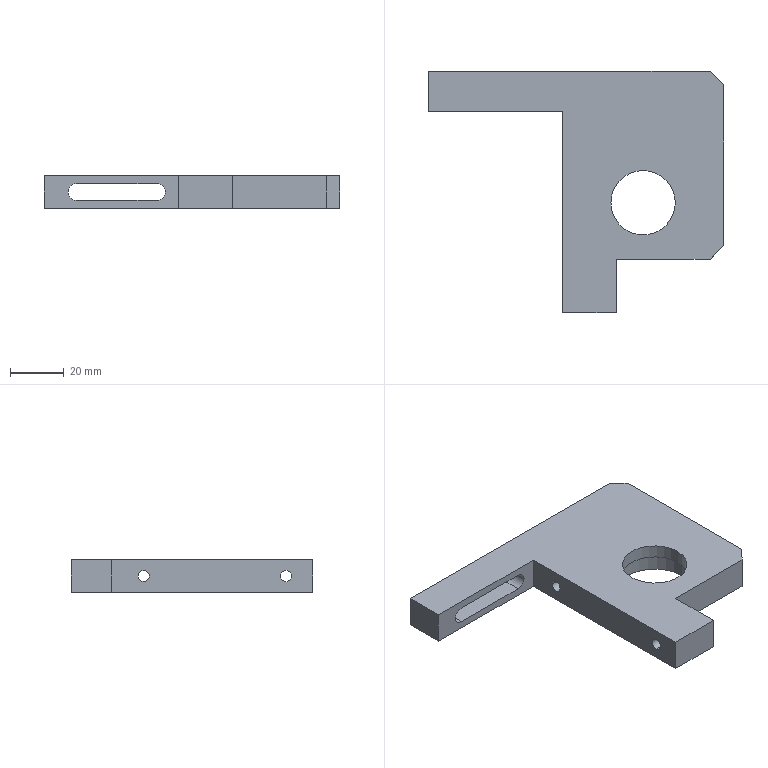Component | SolidWorks | LD101-02--Q1025-Q1-2-1 | 1 solid | 29 faces | box 110 x 90 x 12 mm | volume 50389 mm3 | plane 16 | cylinder 13 | commonest cylinder face diameters 4.2 x4 6.2 x3 10 x2 24 x2 28 x2 | material 45
build123d program:
from build123d import *

# Parameters (mm, degrees)
SKETCH1_W           = 110
SKETCH1_H           = 90
BOSS_EXTRUDE1_DEPTH = 6
SKETCH2_W           = 50
SKETCH2_H           = 75
CUT_EXTRUDE1_DEPTH  = 107.156
SKETCH3_R           = 14
CUT_EXTRUDE2_DEPTH  = 7
SKETCH4_R           = 12
CUT_EXTRUDE3_DEPTH  = 106.707
CUT_EXTRUDE4_DEPTH  = 94.199
SKETCH6_W           = 40
SKETCH6_H           = 20
CUT_EXTRUDE5_DEPTH  = 107.156
M5_TAPPED_HOLE1_D   = 4.2
CHAMFER1_SIZE       = 5
SKETCH9_R           = 5
CUT_EXTRUDE6_DEPTH  = 40
M5_TAPPED_HOLE2_D   = 4.2


with BuildPart() as part:
    # Sketch1 → Boss-Extrude1 (new, symmetric)
    with BuildSketch(Plane(origin=(0, 0, 0), x_dir=(0, 0, -1), z_dir=(1, 0, 0))):
        with Locations((0, 45)):
            Rectangle(SKETCH1_W, SKETCH1_H)
    extrude(amount=BOSS_EXTRUDE1_DEPTH, both=True)

    # Sketch2 → Cut-Extrude1 (cut, through all)
    with BuildSketch(Plane(origin=(6, 0, 0), x_dir=(0, 0, -1), z_dir=(1, 0, 0))):
        with Locations((30, 52.5)):
            Rectangle(SKETCH2_W, SKETCH2_H)
    extrude(amount=-CUT_EXTRUDE1_DEPTH, mode=Mode.SUBTRACT)

    # Sketch3 → Cut-Extrude2 (cut)
    with BuildSketch(Plane.ZY.offset(6)):
        with Locations((25, 49)):
            Circle(SKETCH3_R)
    extrude(amount=-CUT_EXTRUDE2_DEPTH, mode=Mode.SUBTRACT)

    # Sketch4 → Cut-Extrude3 (cut, through all)
    with BuildSketch(Plane.ZY.offset(-1)):
        with Locations((25, 49)):
            Circle(SKETCH4_R)
    extrude(amount=-CUT_EXTRUDE3_DEPTH, mode=Mode.SUBTRACT)

    # Sketch5 → Cut-Extrude4 (cut, through all)
    with BuildSketch(Plane(origin=(0, 15, 0), x_dir=(1, 0, 0), z_dir=(0, 1, 0))):
        with BuildLine():
            Line((3.1, 43), (3.1, 13))
            ThreePointArc((3.1, 13), (0, 9.9), (-3.1, 13))
            Line((-3.1, 13), (-3.1, 43))
            ThreePointArc((-3.1, 43), (0, 46.1), (3.1, 43))
        make_face()
    extrude(amount=-CUT_EXTRUDE4_DEPTH, mode=Mode.SUBTRACT)

    # Sketch6 → Cut-Extrude5 (cut, through all)
    with BuildSketch(Plane.ZY.offset(6)):
        with Locations((35, 80)):
            Rectangle(SKETCH6_W, SKETCH6_H)
    extrude(amount=-CUT_EXTRUDE5_DEPTH, mode=Mode.SUBTRACT)

    # M5 Tapped Hole1 (through all)
    with Locations(Plane(origin=(0, 0, 15), x_dir=(-1, 0, 0), z_dir=(0, 0, 1))):
        with Locations((0, -80)):
            Hole(M5_TAPPED_HOLE1_D / 2)

    # Chamfer1
    chamfer1_edges = [part.edges().sort_by_distance(p)[0] for p in [
        (0, 70, 55),
        (0, 0, 55),
    ]]
    chamfer(chamfer1_edges, length=CHAMFER1_SIZE)

    # Sketch9 → Cut-Extrude6 (cut)
    with BuildSketch(Plane.XY.offset(55)):
        with Locations((0, 27)):
            Circle(SKETCH9_R)
    extrude(amount=-CUT_EXTRUDE6_DEPTH, mode=Mode.SUBTRACT)

    # M5 Tapped Hole2 (through all)
    with Locations(Plane(origin=(0, 0, -5), x_dir=(-1, 0, 0), z_dir=(0, 0, -1))):
        with Locations((0, 27)):
            Hole(M5_TAPPED_HOLE2_D / 2)


solid = part.part

# Placed as in the assembly
solid = solid.moved(Location((346.71, -132.897, 287.257), (180, 90, 0)))
STEP:
#1=COLOUR_RGB('',0.7922,0.8196,0.9333);
#2=FILL_AREA_STYLE_COLOUR('',#1);
#3=FILL_AREA_STYLE('',(#2));
#4=SURFACE_STYLE_FILL_AREA(#3);
#5=SURFACE_SIDE_STYLE('',(#4));
#6=SURFACE_STYLE_USAGE(.BOTH.,#5);
#7=PRESENTATION_STYLE_ASSIGNMENT((#6));
#8=CARTESIAN_POINT('',(14.241,-6.378,11.309));
#9=VERTEX_POINT('',#8);
#10=CARTESIAN_POINT('',(14.241,-6.212,11.309));
#11=VERTEX_POINT('',#10);
#12=CARTESIAN_POINT('',(14.241,-6.295,11.309));
#13=DIRECTION('',(1.,0.,-0.));
#14=DIRECTION('',(0.,1.,0.));
#15=AXIS2_PLACEMENT_3D('',#12,#13,#14);
#16=CIRCLE('',#15,0.08268);
#17=EDGE_CURVE('',#9,#11,#16,.T.);
#18=ORIENTED_EDGE('',*,*,#17,.T.);
#19=CARTESIAN_POINT('',(13.453,-6.212,11.309));
#20=VERTEX_POINT('',#19);
#21=CARTESIAN_POINT('',(13.453,-6.212,11.309));
#22=DIRECTION('',(-1.,-0.,0.));
#23=VECTOR('',#22,39.37);
#24=LINE('',#21,#23);
#25=EDGE_CURVE('',#11,#20,#24,.T.);
#26=ORIENTED_EDGE('',*,*,#25,.T.);
#27=CARTESIAN_POINT('',(13.453,-6.378,11.309));
#28=VERTEX_POINT('',#27);
#29=CARTESIAN_POINT('',(13.453,-6.295,11.309));
#30=DIRECTION('',(-1.,-0.,0.));
#31=DIRECTION('',(0.,-1.,0.));
#32=AXIS2_PLACEMENT_3D('',#29,#30,#31);
#33=CIRCLE('',#32,0.08268);
#34=EDGE_CURVE('',#20,#28,#33,.T.);
#35=ORIENTED_EDGE('',*,*,#34,.T.);
#36=CARTESIAN_POINT('',(13.453,-6.378,11.309));
#37=DIRECTION('',(-1.,-0.,0.));
#38=VECTOR('',#37,39.37);
#39=LINE('',#36,#38);
#40=EDGE_CURVE('',#9,#28,#39,.T.);
#41=ORIENTED_EDGE('',*,*,#40,.F.);
#42=EDGE_LOOP('',(#18,#26,#35,#41));
#43=FACE_OUTER_BOUND('',#42,.T.);
#44=CARTESIAN_POINT('',(13.453,-6.295,11.309));
#45=DIRECTION('',(-1.,-0.,0.));
#46=DIRECTION('',(0.,-1.,0.));
#47=AXIS2_PLACEMENT_3D('',#44,#45,#46);
#48=CYLINDRICAL_SURFACE('',#47,0.08268);
#49=ADVANCED_FACE('',(#43),#48,.F.);
#50=CARTESIAN_POINT('',(14.241,-6.295,11.506));
#51=VERTEX_POINT('',#50);
#52=CARTESIAN_POINT('',(14.241,-6.295,11.112));
#53=VERTEX_POINT('',#52);
#54=CARTESIAN_POINT('',(14.241,-6.295,11.309));
#55=DIRECTION('',(-1.,-0.,0.));
#56=DIRECTION('',(0.,1.,0.));
#57=AXIS2_PLACEMENT_3D('',#54,#55,#56);
#58=CIRCLE('',#57,0.1969);
#59=EDGE_CURVE('',#51,#53,#58,.T.);
#60=ORIENTED_EDGE('',*,*,#59,.T.);
#61=CARTESIAN_POINT('',(15.815,-6.295,11.112));
#62=VERTEX_POINT('',#61);
#63=CARTESIAN_POINT('',(12.896,-6.295,11.112));
#64=DIRECTION('',(1.,0.,-0.));
#65=VECTOR('',#64,39.37);
#66=LINE('',#63,#65);
#67=EDGE_CURVE('',#53,#62,#66,.T.);
#68=ORIENTED_EDGE('',*,*,#67,.T.);
#69=CARTESIAN_POINT('',(15.815,-6.295,11.506));
#70=VERTEX_POINT('',#69);
#71=CARTESIAN_POINT('',(15.815,-6.295,11.309));
#72=DIRECTION('',(1.,0.,-0.));
#73=DIRECTION('',(0.,0.,1.));
#74=AXIS2_PLACEMENT_3D('',#71,#72,#73);
#75=CIRCLE('',#74,0.1969);
#76=EDGE_CURVE('',#62,#70,#75,.T.);
#77=ORIENTED_EDGE('',*,*,#76,.T.);
#78=CARTESIAN_POINT('',(12.896,-6.295,11.506));
#79=DIRECTION('',(1.,0.,-0.));
#80=VECTOR('',#79,39.37);
#81=LINE('',#78,#80);
#82=EDGE_CURVE('',#51,#70,#81,.T.);
#83=ORIENTED_EDGE('',*,*,#82,.F.);
#84=EDGE_LOOP('',(#60,#68,#77,#83));
#85=FACE_OUTER_BOUND('',#84,.T.);
#86=CARTESIAN_POINT('',(12.896,-6.295,11.309));
#87=DIRECTION('',(1.,0.,-0.));
#88=DIRECTION('',(0.,0.,1.));
#89=AXIS2_PLACEMENT_3D('',#86,#87,#88);
#90=CYLINDRICAL_SURFACE('',#89,0.1969);
#91=ADVANCED_FACE('',(#85),#90,.F.);
#92=CARTESIAN_POINT('',(13.453,-8.382,11.227));
#93=VERTEX_POINT('',#92);
#94=CARTESIAN_POINT('',(13.453,-8.382,11.392));
#95=VERTEX_POINT('',#94);
#96=CARTESIAN_POINT('',(13.453,-8.382,11.309));
#97=DIRECTION('',(1.,0.,-0.));
#98=DIRECTION('',(0.,1.,0.));
#99=AXIS2_PLACEMENT_3D('',#96,#97,#98);
#100=CIRCLE('',#99,0.08268);
#101=EDGE_CURVE('',#93,#95,#100,.T.);
#102=ORIENTED_EDGE('',*,*,#101,.F.);
#103=CARTESIAN_POINT('',(14.241,-8.382,11.227));
#104=VERTEX_POINT('',#103);
#105=CARTESIAN_POINT('',(14.241,-8.382,11.227));
#106=DIRECTION('',(1.,0.,-0.));
#107=VECTOR('',#106,39.37);
#108=LINE('',#105,#107);
#109=EDGE_CURVE('',#93,#104,#108,.T.);
#110=ORIENTED_EDGE('',*,*,#109,.T.);
#111=CARTESIAN_POINT('',(14.241,-8.382,11.392));
#112=VERTEX_POINT('',#111);
#113=CARTESIAN_POINT('',(14.241,-8.382,11.309));
#114=DIRECTION('',(1.,0.,-0.));
#115=DIRECTION('',(0.,0.,1.));
#116=AXIS2_PLACEMENT_3D('',#113,#114,#115);
#117=CIRCLE('',#116,0.08268);
#118=EDGE_CURVE('',#104,#112,#117,.T.);
#119=ORIENTED_EDGE('',*,*,#118,.T.);
#120=CARTESIAN_POINT('',(14.241,-8.382,11.392));
#121=DIRECTION('',(1.,0.,-0.));
#122=VECTOR('',#121,39.37);
#123=LINE('',#120,#122);
#124=EDGE_CURVE('',#95,#112,#123,.T.);
#125=ORIENTED_EDGE('',*,*,#124,.F.);
#126=EDGE_LOOP('',(#102,#110,#119,#125));
#127=FACE_OUTER_BOUND('',#126,.T.);
#128=CARTESIAN_POINT('',(14.241,-8.382,11.309));
#129=DIRECTION('',(1.,0.,-0.));
#130=DIRECTION('',(0.,0.,1.));
#131=AXIS2_PLACEMENT_3D('',#128,#129,#130);
#132=CYLINDRICAL_SURFACE('',#131,0.08268);
#133=ADVANCED_FACE('',(#127),#132,.F.);
#134=CARTESIAN_POINT('',(13.26,-5.232,11.309));
#135=VERTEX_POINT('',#134);
#136=CARTESIAN_POINT('',(13.138,-5.232,11.431));
#137=VERTEX_POINT('',#136);
#138=CARTESIAN_POINT('',(13.138,-5.232,11.309));
#139=DIRECTION('',(0.,-1.,0.));
#140=DIRECTION('',(1.,0.,0.));
#141=AXIS2_PLACEMENT_3D('',#138,#139,#140);
#142=CIRCLE('',#141,0.122);
#143=EDGE_CURVE('',#135,#137,#142,.T.);
#144=ORIENTED_EDGE('',*,*,#143,.F.);
#145=CARTESIAN_POINT('',(13.26,-5.823,11.309));
#146=VERTEX_POINT('',#145);
#147=CARTESIAN_POINT('',(13.26,-5.232,11.309));
#148=DIRECTION('',(0.,-1.,0.));
#149=VECTOR('',#148,39.37);
#150=LINE('',#147,#149);
#151=EDGE_CURVE('',#135,#146,#150,.T.);
#152=ORIENTED_EDGE('',*,*,#151,.T.);
#153=CARTESIAN_POINT('',(13.138,-5.823,11.431));
#154=VERTEX_POINT('',#153);
#155=CARTESIAN_POINT('',(13.138,-5.823,11.309));
#156=DIRECTION('',(0.,-1.,0.));
#157=DIRECTION('',(1.,0.,0.));
#158=AXIS2_PLACEMENT_3D('',#155,#156,#157);
#159=CIRCLE('',#158,0.122);
#160=EDGE_CURVE('',#146,#154,#159,.T.);
#161=ORIENTED_EDGE('',*,*,#160,.T.);
#162=CARTESIAN_POINT('',(13.138,-5.232,11.431));
#163=DIRECTION('',(0.,-1.,0.));
#164=VECTOR('',#163,39.37);
#165=LINE('',#162,#164);
#166=EDGE_CURVE('',#137,#154,#165,.T.);
#167=ORIENTED_EDGE('',*,*,#166,.F.);
#168=EDGE_LOOP('',(#144,#152,#161,#167));
#169=FACE_OUTER_BOUND('',#168,.T.);
#170=CARTESIAN_POINT('',(13.138,-5.232,11.309));
#171=DIRECTION('',(0.,-1.,0.));
#172=DIRECTION('',(1.,0.,0.));
#173=AXIS2_PLACEMENT_3D('',#170,#171,#172);
#174=CYLINDRICAL_SURFACE('',#173,0.122);
#175=ADVANCED_FACE('',(#169),#174,.F.);
#176=CARTESIAN_POINT('',(14.162,-7.161,11.546));
#177=VERTEX_POINT('',#176);
#178=CARTESIAN_POINT('',(15.107,-7.161,11.546));
#179=VERTEX_POINT('',#178);
#180=CARTESIAN_POINT('',(14.634,-7.161,11.546));
#181=DIRECTION('',(0.,-0.,-1.));
#182=DIRECTION('',(1.,0.,0.));
#183=AXIS2_PLACEMENT_3D('',#180,#181,#182);
#184=CIRCLE('',#183,0.4724);
#185=EDGE_CURVE('',#177,#179,#184,.T.);
#186=ORIENTED_EDGE('',*,*,#185,.F.);
#187=CARTESIAN_POINT('',(14.162,-7.161,11.349));
#188=VERTEX_POINT('',#187);
#189=CARTESIAN_POINT('',(14.162,-7.161,11.546));
#190=DIRECTION('',(0.,-0.,-1.));
#191=VECTOR('',#190,39.37);
#192=LINE('',#189,#191);
#193=EDGE_CURVE('',#177,#188,#192,.T.);
#194=ORIENTED_EDGE('',*,*,#193,.T.);
#195=CARTESIAN_POINT('',(15.107,-7.161,11.349));
#196=VERTEX_POINT('',#195);
#197=CARTESIAN_POINT('',(14.634,-7.161,11.349));
#198=DIRECTION('',(0.,-0.,-1.));
#199=DIRECTION('',(1.,0.,0.));
#200=AXIS2_PLACEMENT_3D('',#197,#198,#199);
#201=CIRCLE('',#200,0.4724);
#202=EDGE_CURVE('',#188,#196,#201,.T.);
#203=ORIENTED_EDGE('',*,*,#202,.T.);
#204=CARTESIAN_POINT('',(15.107,-7.161,11.546));
#205=DIRECTION('',(0.,-0.,-1.));
#206=VECTOR('',#205,39.37);
#207=LINE('',#204,#206);
#208=EDGE_CURVE('',#179,#196,#207,.T.);
#209=ORIENTED_EDGE('',*,*,#208,.F.);
#210=EDGE_LOOP('',(#186,#194,#203,#209));
#211=FACE_OUTER_BOUND('',#210,.T.);
#212=CARTESIAN_POINT('',(14.634,-7.161,11.546));
#213=DIRECTION('',(0.,-0.,-1.));
#214=DIRECTION('',(1.,0.,0.));
#215=AXIS2_PLACEMENT_3D('',#212,#213,#214);
#216=CYLINDRICAL_SURFACE('',#215,0.4724);
#217=ADVANCED_FACE('',(#211),#216,.F.);
#218=CARTESIAN_POINT('',(14.083,-7.161,11.349));
#219=VERTEX_POINT('',#218);
#220=CARTESIAN_POINT('',(15.185,-7.161,11.349));
#221=VERTEX_POINT('',#220);
#222=CARTESIAN_POINT('',(14.634,-7.161,11.349));
#223=DIRECTION('',(0.,-0.,-1.));
#224=DIRECTION('',(1.,0.,0.));
#225=AXIS2_PLACEMENT_3D('',#222,#223,#224);
#226=CIRCLE('',#225,0.5512);
#227=EDGE_CURVE('',#219,#221,#226,.T.);
#228=ORIENTED_EDGE('',*,*,#227,.F.);
#229=CARTESIAN_POINT('',(14.083,-7.161,11.073));
#230=VERTEX_POINT('',#229);
#231=CARTESIAN_POINT('',(14.083,-7.161,11.349));
#232=DIRECTION('',(0.,-0.,-1.));
#233=VECTOR('',#232,39.37);
#234=LINE('',#231,#233);
#235=EDGE_CURVE('',#219,#230,#234,.T.);
#236=ORIENTED_EDGE('',*,*,#235,.T.);
#237=CARTESIAN_POINT('',(15.185,-7.161,11.073));
#238=VERTEX_POINT('',#237);
#239=CARTESIAN_POINT('',(14.634,-7.161,11.073));
#240=DIRECTION('',(0.,-0.,-1.));
#241=DIRECTION('',(1.,0.,0.));
#242=AXIS2_PLACEMENT_3D('',#239,#240,#241);
#243=CIRCLE('',#242,0.5512);
#244=EDGE_CURVE('',#230,#238,#243,.T.);
#245=ORIENTED_EDGE('',*,*,#244,.T.);
#246=CARTESIAN_POINT('',(15.185,-7.161,11.349));
#247=DIRECTION('',(0.,-0.,-1.));
#248=VECTOR('',#247,39.37);
#249=LINE('',#246,#248);
#250=EDGE_CURVE('',#221,#238,#249,.T.);
#251=ORIENTED_EDGE('',*,*,#250,.F.);
#252=EDGE_LOOP('',(#228,#236,#245,#251));
#253=FACE_OUTER_BOUND('',#252,.T.);
#254=CARTESIAN_POINT('',(14.634,-7.161,11.349));
#255=DIRECTION('',(0.,-0.,-1.));
#256=DIRECTION('',(1.,0.,0.));
#257=AXIS2_PLACEMENT_3D('',#254,#255,#256);
#258=CYLINDRICAL_SURFACE('',#257,0.5512);
#259=ADVANCED_FACE('',(#253),#258,.F.);
#260=CARTESIAN_POINT('',(13.453,-8.382,11.309));
#261=DIRECTION('',(1.,0.,-0.));
#262=DIRECTION('',(0.,1.,0.));
#263=AXIS2_PLACEMENT_3D('',#260,#261,#262);
#264=CIRCLE('',#263,0.08268);
#265=EDGE_CURVE('',#95,#93,#264,.T.);
#266=ORIENTED_EDGE('',*,*,#265,.T.);
#267=ORIENTED_EDGE('',*,*,#101,.T.);
#268=EDGE_LOOP('',(#266,#267));
#269=FACE_BOUND('',#268,.T.);
#270=CARTESIAN_POINT('',(13.453,-8.775,11.546));
#271=VERTEX_POINT('',#270);
#272=CARTESIAN_POINT('',(13.453,-5.823,11.546));
#273=VERTEX_POINT('',#272);
#274=CARTESIAN_POINT('',(13.453,-8.775,11.546));
#275=DIRECTION('',(-0.,1.,-0.));
#276=VECTOR('',#275,39.37);
#277=LINE('',#274,#276);
#278=EDGE_CURVE('',#271,#273,#277,.T.);
#279=ORIENTED_EDGE('',*,*,#278,.T.);
#280=CARTESIAN_POINT('',(13.453,-5.823,11.073));
#281=VERTEX_POINT('',#280);
#282=CARTESIAN_POINT('',(13.453,-5.823,11.073));
#283=DIRECTION('',(0.,0.,1.));
#284=VECTOR('',#283,39.37);
#285=LINE('',#282,#284);
#286=EDGE_CURVE('',#281,#273,#285,.T.);
#287=ORIENTED_EDGE('',*,*,#286,.F.);
#288=CARTESIAN_POINT('',(13.453,-8.775,11.073));
#289=VERTEX_POINT('',#288);
#290=CARTESIAN_POINT('',(13.453,-8.775,11.073));
#291=DIRECTION('',(-0.,1.,-0.));
#292=VECTOR('',#291,39.37);
#293=LINE('',#290,#292);
#294=EDGE_CURVE('',#289,#281,#293,.T.);
#295=ORIENTED_EDGE('',*,*,#294,.F.);
#296=CARTESIAN_POINT('',(13.453,-8.775,11.073));
#297=DIRECTION('',(0.,0.,1.));
#298=VECTOR('',#297,39.37);
#299=LINE('',#296,#298);
#300=EDGE_CURVE('',#289,#271,#299,.T.);
#301=ORIENTED_EDGE('',*,*,#300,.T.);
#302=EDGE_LOOP('',(#279,#287,#295,#301));
#303=FACE_OUTER_BOUND('',#302,.T.);
#304=CARTESIAN_POINT('',(13.453,-6.295,11.309));
#305=DIRECTION('',(-1.,-0.,0.));
#306=DIRECTION('',(0.,-1.,0.));
#307=AXIS2_PLACEMENT_3D('',#304,#305,#306);
#308=CIRCLE('',#307,0.08268);
#309=EDGE_CURVE('',#28,#20,#308,.T.);
#310=ORIENTED_EDGE('',*,*,#309,.F.);
#311=ORIENTED_EDGE('',*,*,#34,.F.);
#312=EDGE_LOOP('',(#310,#311));
#313=FACE_BOUND('',#312,.T.);
#314=CARTESIAN_POINT('',(13.453,-8.775,11.073));
#315=DIRECTION('',(1.,0.,-0.));
#316=DIRECTION('',(-0.,1.,-0.));
#317=AXIS2_PLACEMENT_3D('',#314,#315,#316);
#318=PLANE('',#317);
#319=ADVANCED_FACE('',(#269,#303,#313),#318,.F.);
#320=CARTESIAN_POINT('',(15.815,-6.295,11.309));
#321=DIRECTION('',(1.,0.,-0.));
#322=DIRECTION('',(0.,0.,1.));
#323=AXIS2_PLACEMENT_3D('',#320,#321,#322);
#324=CIRCLE('',#323,0.1969);
#325=EDGE_CURVE('',#70,#62,#324,.T.);
#326=ORIENTED_EDGE('',*,*,#325,.F.);
#327=ORIENTED_EDGE('',*,*,#76,.F.);
#328=EDGE_LOOP('',(#326,#327));
#329=FACE_BOUND('',#328,.T.);
#330=CARTESIAN_POINT('',(15.815,-7.791,11.546));
#331=VERTEX_POINT('',#330);
#332=CARTESIAN_POINT('',(15.815,-5.429,11.546));
#333=VERTEX_POINT('',#332);
#334=CARTESIAN_POINT('',(15.815,-5.232,11.546));
#335=DIRECTION('',(-0.,1.,-0.));
#336=VECTOR('',#335,39.37);
#337=LINE('',#334,#336);
#338=EDGE_CURVE('',#331,#333,#337,.T.);
#339=ORIENTED_EDGE('',*,*,#338,.F.);
#340=CARTESIAN_POINT('',(15.815,-7.791,11.073));
#341=VERTEX_POINT('',#340);
#342=CARTESIAN_POINT('',(15.815,-7.791,11.546));
#343=DIRECTION('',(0.,-0.,-1.));
#344=VECTOR('',#343,39.37);
#345=LINE('',#342,#344);
#346=EDGE_CURVE('',#331,#341,#345,.T.);
#347=ORIENTED_EDGE('',*,*,#346,.T.);
#348=CARTESIAN_POINT('',(15.815,-5.429,11.073));
#349=VERTEX_POINT('',#348);
#350=CARTESIAN_POINT('',(15.815,-5.232,11.073));
#351=DIRECTION('',(-0.,1.,-0.));
#352=VECTOR('',#351,39.37);
#353=LINE('',#350,#352);
#354=EDGE_CURVE('',#341,#349,#353,.T.);
#355=ORIENTED_EDGE('',*,*,#354,.T.);
#356=CARTESIAN_POINT('',(15.815,-5.429,11.546));
#357=DIRECTION('',(0.,0.,1.));
#358=VECTOR('',#357,39.37);
#359=LINE('',#356,#358);
#360=EDGE_CURVE('',#349,#333,#359,.T.);
#361=ORIENTED_EDGE('',*,*,#360,.T.);
#362=EDGE_LOOP('',(#339,#347,#355,#361));
#363=FACE_OUTER_BOUND('',#362,.T.);
#364=CARTESIAN_POINT('',(15.815,-5.232,11.546));
#365=DIRECTION('',(-1.,-0.,0.));
#366=DIRECTION('',(0.,-0.,-1.));
#367=AXIS2_PLACEMENT_3D('',#364,#365,#366);
#368=PLANE('',#367);
#369=ADVANCED_FACE('',(#329,#363),#368,.F.);
#370=CARTESIAN_POINT('',(11.957,-5.232,11.431));
#371=VERTEX_POINT('',#370);
#372=CARTESIAN_POINT('',(11.957,-5.232,11.431));
#373=DIRECTION('',(-1.,-0.,-0.));
#374=VECTOR('',#373,39.37);
#375=LINE('',#372,#374);
#376=EDGE_CURVE('',#137,#371,#375,.T.);
#377=ORIENTED_EDGE('',*,*,#376,.T.);
#378=CARTESIAN_POINT('',(11.957,-5.232,11.187));
#379=VERTEX_POINT('',#378);
#380=CARTESIAN_POINT('',(11.957,-5.232,11.309));
#381=DIRECTION('',(0.,-1.,0.));
#382=DIRECTION('',(1.,0.,0.));
#383=AXIS2_PLACEMENT_3D('',#380,#381,#382);
#384=CIRCLE('',#383,0.122);
#385=EDGE_CURVE('',#371,#379,#384,.T.);
#386=ORIENTED_EDGE('',*,*,#385,.T.);
#387=CARTESIAN_POINT('',(13.138,-5.232,11.187));
#388=VERTEX_POINT('',#387);
#389=CARTESIAN_POINT('',(11.957,-5.232,11.187));
#390=DIRECTION('',(1.,0.,0.));
#391=VECTOR('',#390,39.37);
#392=LINE('',#389,#391);
#393=EDGE_CURVE('',#379,#388,#392,.T.);
#394=ORIENTED_EDGE('',*,*,#393,.T.);
#395=CARTESIAN_POINT('',(13.138,-5.232,11.309));
#396=DIRECTION('',(0.,-1.,0.));
#397=DIRECTION('',(1.,0.,0.));
#398=AXIS2_PLACEMENT_3D('',#395,#396,#397);
#399=CIRCLE('',#398,0.122);
#400=EDGE_CURVE('',#388,#135,#399,.T.);
#401=ORIENTED_EDGE('',*,*,#400,.T.);
#402=ORIENTED_EDGE('',*,*,#143,.T.);
#403=EDGE_LOOP('',(#377,#386,#394,#401,#402));
#404=FACE_BOUND('',#403,.T.);
#405=CARTESIAN_POINT('',(15.619,-5.232,11.546));
#406=VERTEX_POINT('',#405);
#407=CARTESIAN_POINT('',(11.485,-5.232,11.546));
#408=VERTEX_POINT('',#407);
#409=CARTESIAN_POINT('',(15.815,-5.232,11.546));
#410=DIRECTION('',(-1.,-0.,0.));
#411=VECTOR('',#410,39.37);
#412=LINE('',#409,#411);
#413=EDGE_CURVE('',#406,#408,#412,.T.);
#414=ORIENTED_EDGE('',*,*,#413,.F.);
#415=CARTESIAN_POINT('',(15.619,-5.232,11.073));
#416=VERTEX_POINT('',#415);
#417=CARTESIAN_POINT('',(15.619,-5.232,11.546));
#418=DIRECTION('',(0.,-0.,-1.));
#419=VECTOR('',#418,39.37);
#420=LINE('',#417,#419);
#421=EDGE_CURVE('',#406,#416,#420,.T.);
#422=ORIENTED_EDGE('',*,*,#421,.T.);
#423=CARTESIAN_POINT('',(11.485,-5.232,11.073));
#424=VERTEX_POINT('',#423);
#425=CARTESIAN_POINT('',(15.815,-5.232,11.073));
#426=DIRECTION('',(-1.,-0.,0.));
#427=VECTOR('',#426,39.37);
#428=LINE('',#425,#427);
#429=EDGE_CURVE('',#416,#424,#428,.T.);
#430=ORIENTED_EDGE('',*,*,#429,.T.);
#431=CARTESIAN_POINT('',(11.485,-5.232,11.546));
#432=DIRECTION('',(0.,-0.,-1.));
#433=VECTOR('',#432,39.37);
#434=LINE('',#431,#433);
#435=EDGE_CURVE('',#408,#424,#434,.T.);
#436=ORIENTED_EDGE('',*,*,#435,.F.);
#437=EDGE_LOOP('',(#414,#422,#430,#436));
#438=FACE_OUTER_BOUND('',#437,.T.);
#439=CARTESIAN_POINT('',(15.815,-5.232,11.546));
#440=DIRECTION('',(0.,-1.,0.));
#441=DIRECTION('',(1.,0.,-0.));
#442=AXIS2_PLACEMENT_3D('',#439,#440,#441);
#443=PLANE('',#442);
#444=ADVANCED_FACE('',(#404,#438),#443,.F.);
#445=CARTESIAN_POINT('',(11.485,-5.823,11.073));
#446=VERTEX_POINT('',#445);
#447=CARTESIAN_POINT('',(11.485,-5.232,11.073));
#448=DIRECTION('',(0.,-1.,0.));
#449=VECTOR('',#448,39.37);
#450=LINE('',#447,#449);
#451=EDGE_CURVE('',#424,#446,#450,.T.);
#452=ORIENTED_EDGE('',*,*,#451,.T.);
#453=CARTESIAN_POINT('',(11.485,-5.823,11.546));
#454=VERTEX_POINT('',#453);
#455=CARTESIAN_POINT('',(11.485,-5.823,11.073));
#456=DIRECTION('',(0.,0.,1.));
#457=VECTOR('',#456,39.37);
#458=LINE('',#455,#457);
#459=EDGE_CURVE('',#446,#454,#458,.T.);
#460=ORIENTED_EDGE('',*,*,#459,.T.);
#461=CARTESIAN_POINT('',(11.485,-5.232,11.546));
#462=DIRECTION('',(0.,-1.,0.));
#463=VECTOR('',#462,39.37);
#464=LINE('',#461,#463);
#465=EDGE_CURVE('',#408,#454,#464,.T.);
#466=ORIENTED_EDGE('',*,*,#465,.F.);
#467=ORIENTED_EDGE('',*,*,#435,.T.);
#468=EDGE_LOOP('',(#452,#460,#466,#467));
#469=FACE_OUTER_BOUND('',#468,.T.);
#470=CARTESIAN_POINT('',(11.485,-5.232,11.546));
#471=DIRECTION('',(1.,0.,-0.));
#472=DIRECTION('',(0.,0.,1.));
#473=AXIS2_PLACEMENT_3D('',#470,#471,#472);
#474=PLANE('',#473);
#475=ADVANCED_FACE('',(#469),#474,.F.);
#476=CARTESIAN_POINT('',(14.241,-8.775,11.073));
#477=VERTEX_POINT('',#476);
#478=CARTESIAN_POINT('',(15.815,-8.775,11.073));
#479=DIRECTION('',(1.,0.,-0.));
#480=VECTOR('',#479,39.37);
#481=LINE('',#478,#480);
#482=EDGE_CURVE('',#289,#477,#481,.T.);
#483=ORIENTED_EDGE('',*,*,#482,.T.);
#484=CARTESIAN_POINT('',(14.241,-8.775,11.546));
#485=VERTEX_POINT('',#484);
#486=CARTESIAN_POINT('',(14.241,-8.775,11.546));
#487=DIRECTION('',(0.,-0.,-1.));
#488=VECTOR('',#487,39.37);
#489=LINE('',#486,#488);
#490=EDGE_CURVE('',#485,#477,#489,.T.);
#491=ORIENTED_EDGE('',*,*,#490,.F.);
#492=CARTESIAN_POINT('',(15.815,-8.775,11.546));
#493=DIRECTION('',(1.,0.,-0.));
#494=VECTOR('',#493,39.37);
#495=LINE('',#492,#494);
#496=EDGE_CURVE('',#271,#485,#495,.T.);
#497=ORIENTED_EDGE('',*,*,#496,.F.);
#498=ORIENTED_EDGE('',*,*,#300,.F.);
#499=EDGE_LOOP('',(#483,#491,#497,#498));
#500=FACE_OUTER_BOUND('',#499,.T.);
#501=CARTESIAN_POINT('',(15.815,-8.775,11.546));
#502=DIRECTION('',(-0.,1.,-0.));
#503=DIRECTION('',(-1.,-0.,0.));
#504=AXIS2_PLACEMENT_3D('',#501,#502,#503);
#505=PLANE('',#504);
#506=ADVANCED_FACE('',(#500),#505,.F.);
#507=CARTESIAN_POINT('',(14.634,-7.161,11.546));
#508=DIRECTION('',(0.,-0.,-1.));
#509=DIRECTION('',(1.,0.,0.));
#510=AXIS2_PLACEMENT_3D('',#507,#508,#509);
#511=CIRCLE('',#510,0.4724);
#512=EDGE_CURVE('',#179,#177,#511,.T.);
#513=ORIENTED_EDGE('',*,*,#512,.T.);
#514=ORIENTED_EDGE('',*,*,#185,.T.);
#515=EDGE_LOOP('',(#513,#514));
#516=FACE_BOUND('',#515,.T.);
#517=CARTESIAN_POINT('',(14.241,-7.988,11.546));
#518=VERTEX_POINT('',#517);
#519=CARTESIAN_POINT('',(15.619,-7.988,11.546));
#520=VERTEX_POINT('',#519);
#521=CARTESIAN_POINT('',(14.241,-7.988,11.546));
#522=DIRECTION('',(1.,0.,-0.));
#523=VECTOR('',#522,39.37);
#524=LINE('',#521,#523);
#525=EDGE_CURVE('',#518,#520,#524,.T.);
#526=ORIENTED_EDGE('',*,*,#525,.T.);
#527=CARTESIAN_POINT('',(15.815,-7.791,11.546));
#528=DIRECTION('',(0.7071,0.7071,-0.));
#529=VECTOR('',#528,39.37);
#530=LINE('',#527,#529);
#531=EDGE_CURVE('',#520,#331,#530,.T.);
#532=ORIENTED_EDGE('',*,*,#531,.T.);
#533=ORIENTED_EDGE('',*,*,#338,.T.);
#534=CARTESIAN_POINT('',(15.619,-5.232,11.546));
#535=DIRECTION('',(-0.7071,0.7071,-0.));
#536=VECTOR('',#535,39.37);
#537=LINE('',#534,#536);
#538=EDGE_CURVE('',#333,#406,#537,.T.);
#539=ORIENTED_EDGE('',*,*,#538,.T.);
#540=ORIENTED_EDGE('',*,*,#413,.T.);
#541=ORIENTED_EDGE('',*,*,#465,.T.);
#542=CARTESIAN_POINT('',(11.485,-5.823,11.546));
#543=DIRECTION('',(-1.,-0.,0.));
#544=VECTOR('',#543,39.37);
#545=LINE('',#542,#544);
#546=EDGE_CURVE('',#273,#454,#545,.T.);
#547=ORIENTED_EDGE('',*,*,#546,.F.);
#548=ORIENTED_EDGE('',*,*,#278,.F.);
#549=ORIENTED_EDGE('',*,*,#496,.T.);
#550=CARTESIAN_POINT('',(14.241,-8.775,11.546));
#551=DIRECTION('',(0.,1.,-0.));
#552=VECTOR('',#551,39.37);
#553=LINE('',#550,#552);
#554=EDGE_CURVE('',#485,#518,#553,.T.);
#555=ORIENTED_EDGE('',*,*,#554,.T.);
#556=EDGE_LOOP('',(#526,#532,#533,#539,#540,#541,#547,#548,#549,#555));
#557=FACE_OUTER_BOUND('',#556,.T.);
#558=CARTESIAN_POINT('',(13.65,-5.232,11.546));
#559=DIRECTION('',(-0.,-0.,-1.));
#560=DIRECTION('',(1.,0.,-0.));
#561=AXIS2_PLACEMENT_3D('',#558,#559,#560);
#562=PLANE('',#561);
#563=ADVANCED_FACE('',(#516,#557),#562,.F.);
#564=ORIENTED_EDGE('',*,*,#354,.F.);
#565=CARTESIAN_POINT('',(15.619,-7.988,11.073));
#566=VERTEX_POINT('',#565);
#567=CARTESIAN_POINT('',(16.012,-7.594,11.073));
#568=DIRECTION('',(-0.7071,-0.7071,0.));
#569=VECTOR('',#568,39.37);
#570=LINE('',#567,#569);
#571=EDGE_CURVE('',#341,#566,#570,.T.);
#572=ORIENTED_EDGE('',*,*,#571,.T.);
#573=CARTESIAN_POINT('',(14.241,-7.988,11.073));
#574=VERTEX_POINT('',#573);
#575=CARTESIAN_POINT('',(14.241,-7.988,11.073));
#576=DIRECTION('',(1.,0.,-0.));
#577=VECTOR('',#576,39.37);
#578=LINE('',#575,#577);
#579=EDGE_CURVE('',#574,#566,#578,.T.);
#580=ORIENTED_EDGE('',*,*,#579,.F.);
#581=CARTESIAN_POINT('',(14.241,-8.775,11.073));
#582=DIRECTION('',(0.,1.,-0.));
#583=VECTOR('',#582,39.37);
#584=LINE('',#581,#583);
#585=EDGE_CURVE('',#477,#574,#584,.T.);
#586=ORIENTED_EDGE('',*,*,#585,.F.);
#587=ORIENTED_EDGE('',*,*,#482,.F.);
#588=ORIENTED_EDGE('',*,*,#294,.T.);
#589=CARTESIAN_POINT('',(11.485,-5.823,11.073));
#590=DIRECTION('',(-1.,-0.,0.));
#591=VECTOR('',#590,39.37);
#592=LINE('',#589,#591);
#593=EDGE_CURVE('',#281,#446,#592,.T.);
#594=ORIENTED_EDGE('',*,*,#593,.T.);
#595=ORIENTED_EDGE('',*,*,#451,.F.);
#596=ORIENTED_EDGE('',*,*,#429,.F.);
#597=CARTESIAN_POINT('',(14.634,-4.248,11.073));
#598=DIRECTION('',(0.7071,-0.7071,0.));
#599=VECTOR('',#598,39.37);
#600=LINE('',#597,#599);
#601=EDGE_CURVE('',#416,#349,#600,.T.);
#602=ORIENTED_EDGE('',*,*,#601,.T.);
#603=EDGE_LOOP('',(#564,#572,#580,#586,#587,#588,#594,#595,#596,#602));
#604=FACE_OUTER_BOUND('',#603,.T.);
#605=CARTESIAN_POINT('',(14.634,-7.161,11.073));
#606=DIRECTION('',(0.,-0.,-1.));
#607=DIRECTION('',(1.,0.,0.));
#608=AXIS2_PLACEMENT_3D('',#605,#606,#607);
#609=CIRCLE('',#608,0.5512);
#610=EDGE_CURVE('',#238,#230,#609,.T.);
#611=ORIENTED_EDGE('',*,*,#610,.F.);
#612=ORIENTED_EDGE('',*,*,#244,.F.);
#613=EDGE_LOOP('',(#611,#612));
#614=FACE_BOUND('',#613,.T.);
#615=CARTESIAN_POINT('',(13.65,-5.232,11.073));
#616=DIRECTION('',(-0.,-0.,-1.));
#617=DIRECTION('',(1.,0.,-0.));
#618=AXIS2_PLACEMENT_3D('',#615,#616,#617);
#619=PLANE('',#618);
#620=ADVANCED_FACE('',(#604,#614),#619,.T.);
#621=CARTESIAN_POINT('',(11.957,-5.823,11.187));
#622=VERTEX_POINT('',#621);
#623=CARTESIAN_POINT('',(13.138,-5.823,11.187));
#624=VERTEX_POINT('',#623);
#625=CARTESIAN_POINT('',(11.957,-5.823,11.187));
#626=DIRECTION('',(1.,0.,0.));
#627=VECTOR('',#626,39.37);
#628=LINE('',#625,#627);
#629=EDGE_CURVE('',#622,#624,#628,.T.);
#630=ORIENTED_EDGE('',*,*,#629,.F.);
#631=CARTESIAN_POINT('',(11.957,-5.823,11.431));
#632=VERTEX_POINT('',#631);
#633=CARTESIAN_POINT('',(11.957,-5.823,11.309));
#634=DIRECTION('',(0.,-1.,0.));
#635=DIRECTION('',(1.,0.,0.));
#636=AXIS2_PLACEMENT_3D('',#633,#634,#635);
#637=CIRCLE('',#636,0.122);
#638=EDGE_CURVE('',#632,#622,#637,.T.);
#639=ORIENTED_EDGE('',*,*,#638,.F.);
#640=CARTESIAN_POINT('',(11.957,-5.823,11.431));
#641=DIRECTION('',(-1.,-0.,-0.));
#642=VECTOR('',#641,39.37);
#643=LINE('',#640,#642);
#644=EDGE_CURVE('',#154,#632,#643,.T.);
#645=ORIENTED_EDGE('',*,*,#644,.F.);
#646=ORIENTED_EDGE('',*,*,#160,.F.);
#647=CARTESIAN_POINT('',(13.138,-5.823,11.309));
#648=DIRECTION('',(0.,-1.,0.));
#649=DIRECTION('',(1.,0.,0.));
#650=AXIS2_PLACEMENT_3D('',#647,#648,#649);
#651=CIRCLE('',#650,0.122);
#652=EDGE_CURVE('',#624,#146,#651,.T.);
#653=ORIENTED_EDGE('',*,*,#652,.F.);
#654=EDGE_LOOP('',(#630,#639,#645,#646,#653));
#655=FACE_BOUND('',#654,.T.);
#656=ORIENTED_EDGE('',*,*,#546,.T.);
#657=ORIENTED_EDGE('',*,*,#459,.F.);
#658=ORIENTED_EDGE('',*,*,#593,.F.);
#659=ORIENTED_EDGE('',*,*,#286,.T.);
#660=EDGE_LOOP('',(#656,#657,#658,#659));
#661=FACE_OUTER_BOUND('',#660,.T.);
#662=CARTESIAN_POINT('',(11.485,-5.823,11.073));
#663=DIRECTION('',(-0.,1.,-0.));
#664=DIRECTION('',(-1.,-0.,0.));
#665=AXIS2_PLACEMENT_3D('',#662,#663,#664);
#666=PLANE('',#665);
#667=ADVANCED_FACE('',(#655,#661),#666,.F.);
#668=ORIENTED_EDGE('',*,*,#235,.F.);
#669=CARTESIAN_POINT('',(14.634,-7.161,11.349));
#670=DIRECTION('',(0.,-0.,-1.));
#671=DIRECTION('',(1.,0.,0.));
#672=AXIS2_PLACEMENT_3D('',#669,#670,#671);
#673=CIRCLE('',#672,0.5512);
#674=EDGE_CURVE('',#221,#219,#673,.T.);
#675=ORIENTED_EDGE('',*,*,#674,.F.);
#676=ORIENTED_EDGE('',*,*,#250,.T.);
#677=ORIENTED_EDGE('',*,*,#610,.T.);
#678=EDGE_LOOP('',(#668,#675,#676,#677));
#679=FACE_OUTER_BOUND('',#678,.T.);
#680=CARTESIAN_POINT('',(14.634,-7.161,11.349));
#681=DIRECTION('',(0.,-0.,-1.));
#682=DIRECTION('',(1.,0.,0.));
#683=AXIS2_PLACEMENT_3D('',#680,#681,#682);
#684=CYLINDRICAL_SURFACE('',#683,0.5512);
#685=ADVANCED_FACE('',(#679),#684,.F.);
#686=CARTESIAN_POINT('',(14.634,-7.161,11.349));
#687=DIRECTION('',(0.,-0.,-1.));
#688=DIRECTION('',(1.,0.,0.));
#689=AXIS2_PLACEMENT_3D('',#686,#687,#688);
#690=CIRCLE('',#689,0.4724);
#691=EDGE_CURVE('',#196,#188,#690,.T.);
#692=ORIENTED_EDGE('',*,*,#691,.F.);
#693=ORIENTED_EDGE('',*,*,#202,.F.);
#694=EDGE_LOOP('',(#692,#693));
#695=FACE_BOUND('',#694,.T.);
#696=ORIENTED_EDGE('',*,*,#674,.T.);
#697=ORIENTED_EDGE('',*,*,#227,.T.);
#698=EDGE_LOOP('',(#696,#697));
#699=FACE_OUTER_BOUND('',#698,.T.);
#700=CARTESIAN_POINT('',(14.634,-7.161,11.349));
#701=DIRECTION('',(-0.,-0.,-1.));
#702=DIRECTION('',(1.,0.,-0.));
#703=AXIS2_PLACEMENT_3D('',#700,#701,#702);
#704=PLANE('',#703);
#705=ADVANCED_FACE('',(#695,#699),#704,.T.);
#706=ORIENTED_EDGE('',*,*,#193,.F.);
#707=ORIENTED_EDGE('',*,*,#512,.F.);
#708=ORIENTED_EDGE('',*,*,#208,.T.);
#709=ORIENTED_EDGE('',*,*,#691,.T.);
#710=EDGE_LOOP('',(#706,#707,#708,#709));
#711=FACE_OUTER_BOUND('',#710,.T.);
#712=CARTESIAN_POINT('',(14.634,-7.161,11.546));
#713=DIRECTION('',(0.,-0.,-1.));
#714=DIRECTION('',(1.,0.,0.));
#715=AXIS2_PLACEMENT_3D('',#712,#713,#714);
#716=CYLINDRICAL_SURFACE('',#715,0.4724);
#717=ADVANCED_FACE('',(#711),#716,.F.);
#718=ORIENTED_EDGE('',*,*,#638,.T.);
#719=CARTESIAN_POINT('',(11.957,-5.232,11.187));
#720=DIRECTION('',(0.,-1.,0.));
#721=VECTOR('',#720,39.37);
#722=LINE('',#719,#721);
#723=EDGE_CURVE('',#379,#622,#722,.T.);
#724=ORIENTED_EDGE('',*,*,#723,.F.);
#725=ORIENTED_EDGE('',*,*,#385,.F.);
#726=CARTESIAN_POINT('',(11.957,-5.232,11.431));
#727=DIRECTION('',(0.,-1.,0.));
#728=VECTOR('',#727,39.37);
#729=LINE('',#726,#728);
#730=EDGE_CURVE('',#371,#632,#729,.T.);
#731=ORIENTED_EDGE('',*,*,#730,.T.);
#732=EDGE_LOOP('',(#718,#724,#725,#731));
#733=FACE_OUTER_BOUND('',#732,.T.);
#734=CARTESIAN_POINT('',(11.957,-5.232,11.309));
#735=DIRECTION('',(0.,-1.,0.));
#736=DIRECTION('',(1.,0.,0.));
#737=AXIS2_PLACEMENT_3D('',#734,#735,#736);
#738=CYLINDRICAL_SURFACE('',#737,0.122);
#739=ADVANCED_FACE('',(#733),#738,.F.);
#740=ORIENTED_EDGE('',*,*,#644,.T.);
#741=ORIENTED_EDGE('',*,*,#730,.F.);
#742=ORIENTED_EDGE('',*,*,#376,.F.);
#743=ORIENTED_EDGE('',*,*,#166,.T.);
#744=EDGE_LOOP('',(#740,#741,#742,#743));
#745=FACE_OUTER_BOUND('',#744,.T.);
#746=CARTESIAN_POINT('',(11.957,-5.232,11.431));
#747=DIRECTION('',(-0.,0.,1.));
#748=DIRECTION('',(-1.,-0.,-0.));
#749=AXIS2_PLACEMENT_3D('',#746,#747,#748);
#750=PLANE('',#749);
#751=ADVANCED_FACE('',(#745),#750,.F.);
#752=ORIENTED_EDGE('',*,*,#151,.F.);
#753=ORIENTED_EDGE('',*,*,#400,.F.);
#754=CARTESIAN_POINT('',(13.138,-5.232,11.187));
#755=DIRECTION('',(0.,-1.,0.));
#756=VECTOR('',#755,39.37);
#757=LINE('',#754,#756);
#758=EDGE_CURVE('',#388,#624,#757,.T.);
#759=ORIENTED_EDGE('',*,*,#758,.T.);
#760=ORIENTED_EDGE('',*,*,#652,.T.);
#761=EDGE_LOOP('',(#752,#753,#759,#760));
#762=FACE_OUTER_BOUND('',#761,.T.);
#763=CARTESIAN_POINT('',(13.138,-5.232,11.309));
#764=DIRECTION('',(0.,-1.,0.));
#765=DIRECTION('',(1.,0.,0.));
#766=AXIS2_PLACEMENT_3D('',#763,#764,#765);
#767=CYLINDRICAL_SURFACE('',#766,0.122);
#768=ADVANCED_FACE('',(#762),#767,.F.);
#769=ORIENTED_EDGE('',*,*,#629,.T.);
#770=ORIENTED_EDGE('',*,*,#758,.F.);
#771=ORIENTED_EDGE('',*,*,#393,.F.);
#772=ORIENTED_EDGE('',*,*,#723,.T.);
#773=EDGE_LOOP('',(#769,#770,#771,#772));
#774=FACE_OUTER_BOUND('',#773,.T.);
#775=CARTESIAN_POINT('',(11.957,-5.232,11.187));
#776=DIRECTION('',(0.,-0.,-1.));
#777=DIRECTION('',(1.,0.,0.));
#778=AXIS2_PLACEMENT_3D('',#775,#776,#777);
#779=PLANE('',#778);
#780=ADVANCED_FACE('',(#774),#779,.F.);
#781=CARTESIAN_POINT('',(14.241,-8.382,11.309));
#782=DIRECTION('',(1.,0.,-0.));
#783=DIRECTION('',(0.,0.,1.));
#784=AXIS2_PLACEMENT_3D('',#781,#782,#783);
#785=CIRCLE('',#784,0.08268);
#786=EDGE_CURVE('',#112,#104,#785,.T.);
#787=ORIENTED_EDGE('',*,*,#786,.F.);
#788=ORIENTED_EDGE('',*,*,#118,.F.);
#789=EDGE_LOOP('',(#787,#788));
#790=FACE_BOUND('',#789,.T.);
#791=ORIENTED_EDGE('',*,*,#585,.T.);
#792=CARTESIAN_POINT('',(14.241,-7.988,11.546));
#793=DIRECTION('',(0.,-0.,-1.));
#794=VECTOR('',#793,39.37);
#795=LINE('',#792,#794);
#796=EDGE_CURVE('',#518,#574,#795,.T.);
#797=ORIENTED_EDGE('',*,*,#796,.F.);
#798=ORIENTED_EDGE('',*,*,#554,.F.);
#799=ORIENTED_EDGE('',*,*,#490,.T.);
#800=EDGE_LOOP('',(#791,#797,#798,#799));
#801=FACE_OUTER_BOUND('',#800,.T.);
#802=CARTESIAN_POINT('',(14.241,-8.775,11.546));
#803=DIRECTION('',(-1.,0.,0.));
#804=DIRECTION('',(-0.,-1.,0.));
#805=AXIS2_PLACEMENT_3D('',#802,#803,#804);
#806=PLANE('',#805);
#807=ADVANCED_FACE('',(#790,#801),#806,.F.);
#808=ORIENTED_EDGE('',*,*,#579,.T.);
#809=CARTESIAN_POINT('',(15.619,-7.988,11.546));
#810=DIRECTION('',(0.,0.,1.));
#811=VECTOR('',#810,39.37);
#812=LINE('',#809,#811);
#813=EDGE_CURVE('',#566,#520,#812,.T.);
#814=ORIENTED_EDGE('',*,*,#813,.T.);
#815=ORIENTED_EDGE('',*,*,#525,.F.);
#816=ORIENTED_EDGE('',*,*,#796,.T.);
#817=EDGE_LOOP('',(#808,#814,#815,#816));
#818=FACE_OUTER_BOUND('',#817,.T.);
#819=CARTESIAN_POINT('',(14.241,-7.988,11.546));
#820=DIRECTION('',(-0.,1.,-0.));
#821=DIRECTION('',(-1.,-0.,0.));
#822=AXIS2_PLACEMENT_3D('',#819,#820,#821);
#823=PLANE('',#822);
#824=ADVANCED_FACE('',(#818),#823,.F.);
#825=ORIENTED_EDGE('',*,*,#109,.F.);
#826=ORIENTED_EDGE('',*,*,#265,.F.);
#827=ORIENTED_EDGE('',*,*,#124,.T.);
#828=ORIENTED_EDGE('',*,*,#786,.T.);
#829=EDGE_LOOP('',(#825,#826,#827,#828));
#830=FACE_OUTER_BOUND('',#829,.T.);
#831=CARTESIAN_POINT('',(14.241,-8.382,11.309));
#832=DIRECTION('',(1.,0.,-0.));
#833=DIRECTION('',(0.,0.,1.));
#834=AXIS2_PLACEMENT_3D('',#831,#832,#833);
#835=CYLINDRICAL_SURFACE('',#834,0.08268);
#836=ADVANCED_FACE('',(#830),#835,.F.);
#837=ORIENTED_EDGE('',*,*,#531,.F.);
#838=ORIENTED_EDGE('',*,*,#813,.F.);
#839=ORIENTED_EDGE('',*,*,#571,.F.);
#840=ORIENTED_EDGE('',*,*,#346,.F.);
#841=EDGE_LOOP('',(#837,#838,#839,#840));
#842=FACE_OUTER_BOUND('',#841,.T.);
#843=CARTESIAN_POINT('',(15.815,-7.791,11.546));
#844=DIRECTION('',(-0.7071,0.7071,-0.));
#845=DIRECTION('',(0.,-0.,-1.));
#846=AXIS2_PLACEMENT_3D('',#843,#844,#845);
#847=PLANE('',#846);
#848=ADVANCED_FACE('',(#842),#847,.F.);
#849=ORIENTED_EDGE('',*,*,#538,.F.);
#850=ORIENTED_EDGE('',*,*,#360,.F.);
#851=ORIENTED_EDGE('',*,*,#601,.F.);
#852=ORIENTED_EDGE('',*,*,#421,.F.);
#853=EDGE_LOOP('',(#849,#850,#851,#852));
#854=FACE_OUTER_BOUND('',#853,.T.);
#855=CARTESIAN_POINT('',(15.619,-5.232,11.546));
#856=DIRECTION('',(-0.7071,-0.7071,0.));
#857=DIRECTION('',(0.,-0.,-1.));
#858=AXIS2_PLACEMENT_3D('',#855,#856,#857);
#859=PLANE('',#858);
#860=ADVANCED_FACE('',(#854),#859,.F.);
#861=ORIENTED_EDGE('',*,*,#67,.F.);
#862=CARTESIAN_POINT('',(14.241,-6.295,11.309));
#863=DIRECTION('',(-1.,-0.,0.));
#864=DIRECTION('',(0.,1.,0.));
#865=AXIS2_PLACEMENT_3D('',#862,#863,#864);
#866=CIRCLE('',#865,0.1969);
#867=EDGE_CURVE('',#53,#51,#866,.T.);
#868=ORIENTED_EDGE('',*,*,#867,.T.);
#869=ORIENTED_EDGE('',*,*,#82,.T.);
#870=ORIENTED_EDGE('',*,*,#325,.T.);
#871=EDGE_LOOP('',(#861,#868,#869,#870));
#872=FACE_OUTER_BOUND('',#871,.T.);
#873=CARTESIAN_POINT('',(12.896,-6.295,11.309));
#874=DIRECTION('',(1.,0.,-0.));
#875=DIRECTION('',(0.,0.,1.));
#876=AXIS2_PLACEMENT_3D('',#873,#874,#875);
#877=CYLINDRICAL_SURFACE('',#876,0.1969);
#878=ADVANCED_FACE('',(#872),#877,.F.);
#879=ORIENTED_EDGE('',*,*,#17,.F.);
#880=CARTESIAN_POINT('',(14.241,-6.295,11.309));
#881=DIRECTION('',(1.,0.,-0.));
#882=DIRECTION('',(0.,1.,0.));
#883=AXIS2_PLACEMENT_3D('',#880,#881,#882);
#884=CIRCLE('',#883,0.08268);
#885=EDGE_CURVE('',#11,#9,#884,.T.);
#886=ORIENTED_EDGE('',*,*,#885,.F.);
#887=EDGE_LOOP('',(#879,#886));
#888=FACE_BOUND('',#887,.T.);
#889=ORIENTED_EDGE('',*,*,#59,.F.);
#890=ORIENTED_EDGE('',*,*,#867,.F.);
#891=EDGE_LOOP('',(#889,#890));
#892=FACE_OUTER_BOUND('',#891,.T.);
#893=CARTESIAN_POINT('',(14.241,-8.775,11.073));
#894=DIRECTION('',(1.,0.,-0.));
#895=DIRECTION('',(-0.,1.,-0.));
#896=AXIS2_PLACEMENT_3D('',#893,#894,#895);
#897=PLANE('',#896);
#898=ADVANCED_FACE('',(#888,#892),#897,.T.);
#899=ORIENTED_EDGE('',*,*,#25,.F.);
#900=ORIENTED_EDGE('',*,*,#885,.T.);
#901=ORIENTED_EDGE('',*,*,#40,.T.);
#902=ORIENTED_EDGE('',*,*,#309,.T.);
#903=EDGE_LOOP('',(#899,#900,#901,#902));
#904=FACE_OUTER_BOUND('',#903,.T.);
#905=CARTESIAN_POINT('',(13.453,-6.295,11.309));
#906=DIRECTION('',(-1.,-0.,0.));
#907=DIRECTION('',(0.,-1.,0.));
#908=AXIS2_PLACEMENT_3D('',#905,#906,#907);
#909=CYLINDRICAL_SURFACE('',#908,0.08268);
#910=ADVANCED_FACE('',(#904),#909,.F.);
#911=CLOSED_SHELL('',(#49,#91,#133,#175,#217,#259,#319,#369,#444,#475,#506,#563,#620,#667,#685,#705,#717,#739,#751,#768,#780,#807,#824,#836,#848,#860,#878,#898,#910));
#912=MANIFOLD_SOLID_BREP('',#911);
#913=STYLED_ITEM('',(#7),#912);
#914=PRESENTATION_LAYER_ASSIGNMENT('','',(#913));
#915=CARTESIAN_POINT('',(0.,0.,0.));
#916=DIRECTION('',(0.,0.,1.));
#917=DIRECTION('',(1.,0.,0.));
#918=AXIS2_PLACEMENT_3D('',#915,#916,#917);
#919=(LENGTH_UNIT()NAMED_UNIT(*)SI_UNIT($,.METRE.));
#920=LENGTH_MEASURE_WITH_UNIT(LENGTH_MEASURE(0.0254),#919);
#921=DIMENSIONAL_EXPONENTS(1.,0.,0.,0.,0.,0.,0.);
#922=(CONVERSION_BASED_UNIT('',#920)LENGTH_UNIT()NAMED_UNIT(#921));
#923=UNCERTAINTY_MEASURE_WITH_UNIT(LENGTH_MEASURE(0.00001),#922,'','');
#924=(NAMED_UNIT(*)PLANE_ANGLE_UNIT()SI_UNIT($,.RADIAN.));
#925=(NAMED_UNIT(*)SI_UNIT($,.STERADIAN.)SOLID_ANGLE_UNIT());
#926=(GEOMETRIC_REPRESENTATION_CONTEXT(3)GLOBAL_UNCERTAINTY_ASSIGNED_CONTEXT((#923))GLOBAL_UNIT_ASSIGNED_CONTEXT((#922,#924,#925))REPRESENTATION_CONTEXT('',''));
#927=ADVANCED_BREP_SHAPE_REPRESENTATION('',(#912,#918),#926);
#928=(LENGTH_UNIT()NAMED_UNIT(*)SI_UNIT($,.METRE.));
#929=LENGTH_MEASURE_WITH_UNIT(LENGTH_MEASURE(0.0254),#928);
#930=DIMENSIONAL_EXPONENTS(1.,0.,0.,0.,0.,0.,0.);
#931=(CONVERSION_BASED_UNIT('',#929)LENGTH_UNIT()NAMED_UNIT(#930));
#932=UNCERTAINTY_MEASURE_WITH_UNIT(LENGTH_MEASURE(0.00001),#931,'','');
#933=(NAMED_UNIT(*)PLANE_ANGLE_UNIT()SI_UNIT($,.RADIAN.));
#934=(NAMED_UNIT(*)SI_UNIT($,.STERADIAN.)SOLID_ANGLE_UNIT());
#935=(GEOMETRIC_REPRESENTATION_CONTEXT(3)GLOBAL_UNCERTAINTY_ASSIGNED_CONTEXT((#932))GLOBAL_UNIT_ASSIGNED_CONTEXT((#931,#933,#934))REPRESENTATION_CONTEXT('',''));
#936=MECHANICAL_DESIGN_GEOMETRIC_PRESENTATION_REPRESENTATION('',(#913),#935);